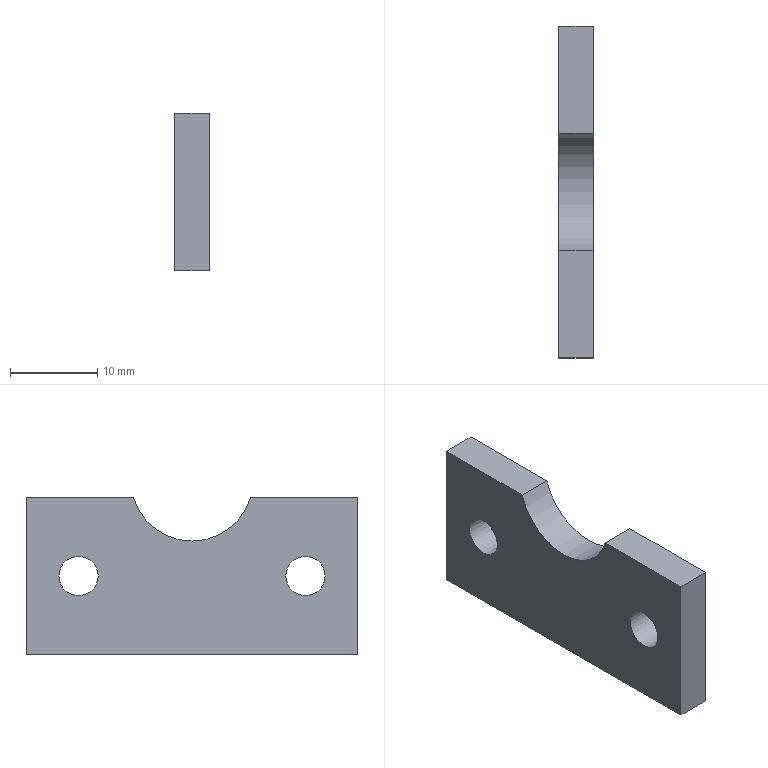Component | NX | BAFFLE_PLATE | 1 solid | 10 faces | box 4 x 38 x 18 mm | volume 2411 mm3 | plane 7 | cylinder 3 | commonest cylinder face diameters 4.5 x2 14 x1
STEP:
#1=CARTESIAN_POINT('',(0.,0.,0.));
#2=DIRECTION('',(0.,0.,1.));
#3=DIRECTION('',(1.,0.,0.));
#4=AXIS2_PLACEMENT_3D('',#1,#2,#3);
#5=CARTESIAN_POINT('',(-20.,-19.,34.5));
#6=VERTEX_POINT('',#5);
#7=CARTESIAN_POINT('',(-20.,-19.,16.5));
#8=VERTEX_POINT('',#7);
#9=CARTESIAN_POINT('',(-20.,-19.,34.5));
#10=DIRECTION('',(0.,0.,-1.));
#11=VECTOR('',#10,1.);
#12=LINE('',#9,#11);
#13=CARTESIAN_POINT('',(-16.,-19.,34.5));
#14=DIRECTION('',(0.,1.,0.));
#15=DIRECTION('',(0.,0.,1.));
#16=AXIS2_PLACEMENT_3D('',#13,#14,#15);
#17=PLANE('',#16);
#18=CARTESIAN_POINT('',(0.,-4.));
#19=DIRECTION('',(-1.,0.));
#20=VECTOR('',#19,1.);
#21=LINE('',#18,#20);
#22=(GEOMETRIC_REPRESENTATION_CONTEXT(2)PARAMETRIC_REPRESENTATION_CONTEXT()REPRESENTATION_CONTEXT('',''));
#23=DEFINITIONAL_REPRESENTATION('',(#21),#22);
#24=PCURVE('',#17,#23);
#25=CARTESIAN_POINT('',(-20.,0.,36.5));
#26=DIRECTION('',(-1.,0.,0.));
#27=DIRECTION('',(0.,0.,1.));
#28=AXIS2_PLACEMENT_3D('',#25,#26,#27);
#29=PLANE('',#28);
#30=CARTESIAN_POINT('',(-2.,-19.));
#31=DIRECTION('',(-1.,0.));
#32=VECTOR('',#31,1.);
#33=LINE('',#30,#32);
#34=(GEOMETRIC_REPRESENTATION_CONTEXT(2)PARAMETRIC_REPRESENTATION_CONTEXT()REPRESENTATION_CONTEXT('',''));
#35=DEFINITIONAL_REPRESENTATION('',(#33),#34);
#36=PCURVE('',#29,#35);
#37=SURFACE_CURVE('',#12,(#24,#36),.PCURVE_S1.);
#38=EDGE_CURVE('',#6,#8,#37,.T.);
#39=ORIENTED_EDGE('',*,*,#38,.T.);
#40=CARTESIAN_POINT('',(-16.,-19.,16.5));
#41=VERTEX_POINT('',#40);
#42=CARTESIAN_POINT('',(-16.,-19.,16.5));
#43=DIRECTION('',(-1.,0.,0.));
#44=VECTOR('',#43,1.);
#45=LINE('',#42,#44);
#46=CARTESIAN_POINT('',(-18.,0.));
#47=DIRECTION('',(0.,-1.));
#48=VECTOR('',#47,1.);
#49=LINE('',#46,#48);
#50=(GEOMETRIC_REPRESENTATION_CONTEXT(2)PARAMETRIC_REPRESENTATION_CONTEXT()REPRESENTATION_CONTEXT('',''));
#51=DEFINITIONAL_REPRESENTATION('',(#49),#50);
#52=PCURVE('',#17,#51);
#53=CARTESIAN_POINT('',(-16.,-19.,16.5));
#54=DIRECTION('',(0.,0.,1.));
#55=DIRECTION('',(1.,0.,0.));
#56=AXIS2_PLACEMENT_3D('',#53,#54,#55);
#57=PLANE('',#56);
#58=CARTESIAN_POINT('',(0.,0.));
#59=DIRECTION('',(-1.,0.));
#60=VECTOR('',#59,1.);
#61=LINE('',#58,#60);
#62=(GEOMETRIC_REPRESENTATION_CONTEXT(2)PARAMETRIC_REPRESENTATION_CONTEXT()REPRESENTATION_CONTEXT('',''));
#63=DEFINITIONAL_REPRESENTATION('',(#61),#62);
#64=PCURVE('',#57,#63);
#65=SURFACE_CURVE('',#45,(#52,#64),.PCURVE_S1.);
#66=EDGE_CURVE('',#41,#8,#65,.T.);
#67=ORIENTED_EDGE('',*,*,#66,.F.);
#68=CARTESIAN_POINT('',(-16.,-19.,34.5));
#69=VERTEX_POINT('',#68);
#70=CARTESIAN_POINT('',(-16.,-19.,34.5));
#71=DIRECTION('',(0.,0.,-1.));
#72=VECTOR('',#71,1.);
#73=LINE('',#70,#72);
#74=CARTESIAN_POINT('',(0.,0.));
#75=DIRECTION('',(-1.,0.));
#76=VECTOR('',#75,1.);
#77=LINE('',#74,#76);
#78=(GEOMETRIC_REPRESENTATION_CONTEXT(2)PARAMETRIC_REPRESENTATION_CONTEXT()REPRESENTATION_CONTEXT('',''));
#79=DEFINITIONAL_REPRESENTATION('',(#77),#78);
#80=PCURVE('',#17,#79);
#81=CARTESIAN_POINT('',(-16.,0.,36.5));
#82=DIRECTION('',(-1.,0.,0.));
#83=DIRECTION('',(0.,0.,1.));
#84=AXIS2_PLACEMENT_3D('',#81,#82,#83);
#85=PLANE('',#84);
#86=CARTESIAN_POINT('',(-2.,-19.));
#87=DIRECTION('',(-1.,0.));
#88=VECTOR('',#87,1.);
#89=LINE('',#86,#88);
#90=(GEOMETRIC_REPRESENTATION_CONTEXT(2)PARAMETRIC_REPRESENTATION_CONTEXT()REPRESENTATION_CONTEXT('',''));
#91=DEFINITIONAL_REPRESENTATION('',(#89),#90);
#92=PCURVE('',#85,#91);
#93=SURFACE_CURVE('',#73,(#80,#92),.PCURVE_S1.);
#94=EDGE_CURVE('',#69,#41,#93,.T.);
#95=ORIENTED_EDGE('',*,*,#94,.F.);
#96=CARTESIAN_POINT('',(-16.,-19.,34.5));
#97=DIRECTION('',(-1.,0.,0.));
#98=VECTOR('',#97,1.);
#99=LINE('',#96,#98);
#100=CARTESIAN_POINT('',(0.,0.));
#101=DIRECTION('',(0.,-1.));
#102=VECTOR('',#101,1.);
#103=LINE('',#100,#102);
#104=(GEOMETRIC_REPRESENTATION_CONTEXT(2)PARAMETRIC_REPRESENTATION_CONTEXT()REPRESENTATION_CONTEXT('',''));
#105=DEFINITIONAL_REPRESENTATION('',(#103),#104);
#106=PCURVE('',#17,#105);
#107=CARTESIAN_POINT('',(-16.,-6.708,34.5));
#108=DIRECTION('',(0.,0.,-1.));
#109=DIRECTION('',(-1.,0.,0.));
#110=AXIS2_PLACEMENT_3D('',#107,#108,#109);
#111=PLANE('',#110);
#112=CARTESIAN_POINT('',(0.,-12.292));
#113=DIRECTION('',(1.,0.));
#114=VECTOR('',#113,1.);
#115=LINE('',#112,#114);
#116=(GEOMETRIC_REPRESENTATION_CONTEXT(2)PARAMETRIC_REPRESENTATION_CONTEXT()REPRESENTATION_CONTEXT('',''));
#117=DEFINITIONAL_REPRESENTATION('',(#115),#116);
#118=PCURVE('',#111,#117);
#119=SURFACE_CURVE('',#99,(#106,#118),.PCURVE_S1.);
#120=EDGE_CURVE('',#69,#6,#119,.T.);
#121=ORIENTED_EDGE('',*,*,#120,.T.);
#122=EDGE_LOOP('',(#39,#67,#95,#121));
#123=FACE_BOUND('',#122,.T.);
#124=ADVANCED_FACE('',(#123),#17,.F.);
#125=CARTESIAN_POINT('',(-20.,19.,16.5));
#126=VERTEX_POINT('',#125);
#127=CARTESIAN_POINT('',(-20.,-19.,16.5));
#128=DIRECTION('',(0.,1.,0.));
#129=VECTOR('',#128,1.);
#130=LINE('',#127,#129);
#131=CARTESIAN_POINT('',(-4.,0.));
#132=DIRECTION('',(0.,1.));
#133=VECTOR('',#132,1.);
#134=LINE('',#131,#133);
#135=(GEOMETRIC_REPRESENTATION_CONTEXT(2)PARAMETRIC_REPRESENTATION_CONTEXT()REPRESENTATION_CONTEXT('',''));
#136=DEFINITIONAL_REPRESENTATION('',(#134),#135);
#137=PCURVE('',#57,#136);
#138=CARTESIAN_POINT('',(-20.,-19.));
#139=DIRECTION('',(0.,1.));
#140=VECTOR('',#139,1.);
#141=LINE('',#138,#140);
#142=(GEOMETRIC_REPRESENTATION_CONTEXT(2)PARAMETRIC_REPRESENTATION_CONTEXT()REPRESENTATION_CONTEXT('',''));
#143=DEFINITIONAL_REPRESENTATION('',(#141),#142);
#144=PCURVE('',#29,#143);
#145=SURFACE_CURVE('',#130,(#137,#144),.PCURVE_S1.);
#146=EDGE_CURVE('',#8,#126,#145,.T.);
#147=ORIENTED_EDGE('',*,*,#146,.T.);
#148=CARTESIAN_POINT('',(-16.,19.,16.5));
#149=VERTEX_POINT('',#148);
#150=CARTESIAN_POINT('',(-16.,19.,16.5));
#151=DIRECTION('',(-1.,0.,0.));
#152=VECTOR('',#151,1.);
#153=LINE('',#150,#152);
#154=CARTESIAN_POINT('',(0.,38.));
#155=DIRECTION('',(-1.,0.));
#156=VECTOR('',#155,1.);
#157=LINE('',#154,#156);
#158=(GEOMETRIC_REPRESENTATION_CONTEXT(2)PARAMETRIC_REPRESENTATION_CONTEXT()REPRESENTATION_CONTEXT('',''));
#159=DEFINITIONAL_REPRESENTATION('',(#157),#158);
#160=PCURVE('',#57,#159);
#161=CARTESIAN_POINT('',(-16.,19.,16.5));
#162=DIRECTION('',(0.,-1.,0.));
#163=DIRECTION('',(0.,0.,-1.));
#164=AXIS2_PLACEMENT_3D('',#161,#162,#163);
#165=PLANE('',#164);
#166=CARTESIAN_POINT('',(0.,0.));
#167=DIRECTION('',(0.,-1.));
#168=VECTOR('',#167,1.);
#169=LINE('',#166,#168);
#170=(GEOMETRIC_REPRESENTATION_CONTEXT(2)PARAMETRIC_REPRESENTATION_CONTEXT()REPRESENTATION_CONTEXT('',''));
#171=DEFINITIONAL_REPRESENTATION('',(#169),#170);
#172=PCURVE('',#165,#171);
#173=SURFACE_CURVE('',#153,(#160,#172),.PCURVE_S1.);
#174=EDGE_CURVE('',#149,#126,#173,.T.);
#175=ORIENTED_EDGE('',*,*,#174,.F.);
#176=CARTESIAN_POINT('',(-16.,-19.,16.5));
#177=DIRECTION('',(0.,1.,0.));
#178=VECTOR('',#177,1.);
#179=LINE('',#176,#178);
#180=CARTESIAN_POINT('',(0.,0.));
#181=DIRECTION('',(0.,1.));
#182=VECTOR('',#181,1.);
#183=LINE('',#180,#182);
#184=(GEOMETRIC_REPRESENTATION_CONTEXT(2)PARAMETRIC_REPRESENTATION_CONTEXT()REPRESENTATION_CONTEXT('',''));
#185=DEFINITIONAL_REPRESENTATION('',(#183),#184);
#186=PCURVE('',#57,#185);
#187=CARTESIAN_POINT('',(-20.,-19.));
#188=DIRECTION('',(0.,1.));
#189=VECTOR('',#188,1.);
#190=LINE('',#187,#189);
#191=(GEOMETRIC_REPRESENTATION_CONTEXT(2)PARAMETRIC_REPRESENTATION_CONTEXT()REPRESENTATION_CONTEXT('',''));
#192=DEFINITIONAL_REPRESENTATION('',(#190),#191);
#193=PCURVE('',#85,#192);
#194=SURFACE_CURVE('',#179,(#186,#193),.PCURVE_S1.);
#195=EDGE_CURVE('',#41,#149,#194,.T.);
#196=ORIENTED_EDGE('',*,*,#195,.F.);
#197=ORIENTED_EDGE('',*,*,#66,.T.);
#198=EDGE_LOOP('',(#147,#175,#196,#197));
#199=FACE_BOUND('',#198,.T.);
#200=ADVANCED_FACE('',(#199),#57,.F.);
#201=CARTESIAN_POINT('',(-20.,19.,34.5));
#202=VERTEX_POINT('',#201);
#203=CARTESIAN_POINT('',(-20.,19.,16.5));
#204=DIRECTION('',(0.,0.,1.));
#205=VECTOR('',#204,1.);
#206=LINE('',#203,#205);
#207=CARTESIAN_POINT('',(0.,-4.));
#208=DIRECTION('',(-1.,0.));
#209=VECTOR('',#208,1.);
#210=LINE('',#207,#209);
#211=(GEOMETRIC_REPRESENTATION_CONTEXT(2)PARAMETRIC_REPRESENTATION_CONTEXT()REPRESENTATION_CONTEXT('',''));
#212=DEFINITIONAL_REPRESENTATION('',(#210),#211);
#213=PCURVE('',#165,#212);
#214=CARTESIAN_POINT('',(-20.,19.));
#215=DIRECTION('',(1.,0.));
#216=VECTOR('',#215,1.);
#217=LINE('',#214,#216);
#218=(GEOMETRIC_REPRESENTATION_CONTEXT(2)PARAMETRIC_REPRESENTATION_CONTEXT()REPRESENTATION_CONTEXT('',''));
#219=DEFINITIONAL_REPRESENTATION('',(#217),#218);
#220=PCURVE('',#29,#219);
#221=SURFACE_CURVE('',#206,(#213,#220),.PCURVE_S1.);
#222=EDGE_CURVE('',#126,#202,#221,.T.);
#223=ORIENTED_EDGE('',*,*,#222,.T.);
#224=CARTESIAN_POINT('',(-16.,19.,34.5));
#225=VERTEX_POINT('',#224);
#226=CARTESIAN_POINT('',(-16.,19.,34.5));
#227=DIRECTION('',(-1.,0.,0.));
#228=VECTOR('',#227,1.);
#229=LINE('',#226,#228);
#230=CARTESIAN_POINT('',(-18.,0.));
#231=DIRECTION('',(0.,-1.));
#232=VECTOR('',#231,1.);
#233=LINE('',#230,#232);
#234=(GEOMETRIC_REPRESENTATION_CONTEXT(2)PARAMETRIC_REPRESENTATION_CONTEXT()REPRESENTATION_CONTEXT('',''));
#235=DEFINITIONAL_REPRESENTATION('',(#233),#234);
#236=PCURVE('',#165,#235);
#237=CARTESIAN_POINT('',(-16.,19.,34.5));
#238=DIRECTION('',(0.,0.,-1.));
#239=DIRECTION('',(-1.,0.,0.));
#240=AXIS2_PLACEMENT_3D('',#237,#238,#239);
#241=PLANE('',#240);
#242=CARTESIAN_POINT('',(0.,0.));
#243=DIRECTION('',(1.,0.));
#244=VECTOR('',#243,1.);
#245=LINE('',#242,#244);
#246=(GEOMETRIC_REPRESENTATION_CONTEXT(2)PARAMETRIC_REPRESENTATION_CONTEXT()REPRESENTATION_CONTEXT('',''));
#247=DEFINITIONAL_REPRESENTATION('',(#245),#246);
#248=PCURVE('',#241,#247);
#249=SURFACE_CURVE('',#229,(#236,#248),.PCURVE_S1.);
#250=EDGE_CURVE('',#225,#202,#249,.T.);
#251=ORIENTED_EDGE('',*,*,#250,.F.);
#252=CARTESIAN_POINT('',(-16.,19.,16.5));
#253=DIRECTION('',(0.,0.,1.));
#254=VECTOR('',#253,1.);
#255=LINE('',#252,#254);
#256=CARTESIAN_POINT('',(0.,0.));
#257=DIRECTION('',(-1.,0.));
#258=VECTOR('',#257,1.);
#259=LINE('',#256,#258);
#260=(GEOMETRIC_REPRESENTATION_CONTEXT(2)PARAMETRIC_REPRESENTATION_CONTEXT()REPRESENTATION_CONTEXT('',''));
#261=DEFINITIONAL_REPRESENTATION('',(#259),#260);
#262=PCURVE('',#165,#261);
#263=CARTESIAN_POINT('',(-20.,19.));
#264=DIRECTION('',(1.,0.));
#265=VECTOR('',#264,1.);
#266=LINE('',#263,#265);
#267=(GEOMETRIC_REPRESENTATION_CONTEXT(2)PARAMETRIC_REPRESENTATION_CONTEXT()REPRESENTATION_CONTEXT('',''));
#268=DEFINITIONAL_REPRESENTATION('',(#266),#267);
#269=PCURVE('',#85,#268);
#270=SURFACE_CURVE('',#255,(#262,#269),.PCURVE_S1.);
#271=EDGE_CURVE('',#149,#225,#270,.T.);
#272=ORIENTED_EDGE('',*,*,#271,.F.);
#273=ORIENTED_EDGE('',*,*,#174,.T.);
#274=EDGE_LOOP('',(#223,#251,#272,#273));
#275=FACE_BOUND('',#274,.T.);
#276=ADVANCED_FACE('',(#275),#165,.F.);
#277=CARTESIAN_POINT('',(-20.,6.708,34.5));
#278=VERTEX_POINT('',#277);
#279=CARTESIAN_POINT('',(-20.,19.,34.5));
#280=DIRECTION('',(0.,-1.,0.));
#281=VECTOR('',#280,1.);
#282=LINE('',#279,#281);
#283=CARTESIAN_POINT('',(4.,0.));
#284=DIRECTION('',(0.,-1.));
#285=VECTOR('',#284,1.);
#286=LINE('',#283,#285);
#287=(GEOMETRIC_REPRESENTATION_CONTEXT(2)PARAMETRIC_REPRESENTATION_CONTEXT()REPRESENTATION_CONTEXT('',''));
#288=DEFINITIONAL_REPRESENTATION('',(#286),#287);
#289=PCURVE('',#241,#288);
#290=CARTESIAN_POINT('',(-2.,19.));
#291=DIRECTION('',(0.,-1.));
#292=VECTOR('',#291,1.);
#293=LINE('',#290,#292);
#294=(GEOMETRIC_REPRESENTATION_CONTEXT(2)PARAMETRIC_REPRESENTATION_CONTEXT()REPRESENTATION_CONTEXT('',''));
#295=DEFINITIONAL_REPRESENTATION('',(#293),#294);
#296=PCURVE('',#29,#295);
#297=SURFACE_CURVE('',#282,(#289,#296),.PCURVE_S1.);
#298=EDGE_CURVE('',#202,#278,#297,.T.);
#299=ORIENTED_EDGE('',*,*,#298,.T.);
#300=CARTESIAN_POINT('',(-16.,6.708,34.5));
#301=VERTEX_POINT('',#300);
#302=CARTESIAN_POINT('',(-16.,6.708,34.5));
#303=DIRECTION('',(-1.,0.,0.));
#304=VECTOR('',#303,1.);
#305=LINE('',#302,#304);
#306=CARTESIAN_POINT('',(0.,-12.292));
#307=DIRECTION('',(1.,0.));
#308=VECTOR('',#307,1.);
#309=LINE('',#306,#308);
#310=(GEOMETRIC_REPRESENTATION_CONTEXT(2)PARAMETRIC_REPRESENTATION_CONTEXT()REPRESENTATION_CONTEXT('',''));
#311=DEFINITIONAL_REPRESENTATION('',(#309),#310);
#312=PCURVE('',#241,#311);
#313=CARTESIAN_POINT('',(-16.,0.,36.5));
#314=DIRECTION('',(-1.,0.,0.));
#315=DIRECTION('',(0.,0.,1.));
#316=AXIS2_PLACEMENT_3D('',#313,#314,#315);
#317=CYLINDRICAL_SURFACE('',#316,7.);
#318=CARTESIAN_POINT('',(1.861,0.));
#319=DIRECTION('',(0.,1.));
#320=VECTOR('',#319,1.);
#321=LINE('',#318,#320);
#322=(GEOMETRIC_REPRESENTATION_CONTEXT(2)PARAMETRIC_REPRESENTATION_CONTEXT()REPRESENTATION_CONTEXT('',''));
#323=DEFINITIONAL_REPRESENTATION('',(#321),#322);
#324=PCURVE('',#317,#323);
#325=SURFACE_CURVE('',#305,(#312,#324),.PCURVE_S1.);
#326=EDGE_CURVE('',#301,#278,#325,.T.);
#327=ORIENTED_EDGE('',*,*,#326,.F.);
#328=CARTESIAN_POINT('',(-16.,19.,34.5));
#329=DIRECTION('',(0.,-1.,0.));
#330=VECTOR('',#329,1.);
#331=LINE('',#328,#330);
#332=CARTESIAN_POINT('',(0.,0.));
#333=DIRECTION('',(0.,-1.));
#334=VECTOR('',#333,1.);
#335=LINE('',#332,#334);
#336=(GEOMETRIC_REPRESENTATION_CONTEXT(2)PARAMETRIC_REPRESENTATION_CONTEXT()REPRESENTATION_CONTEXT('',''));
#337=DEFINITIONAL_REPRESENTATION('',(#335),#336);
#338=PCURVE('',#241,#337);
#339=CARTESIAN_POINT('',(-2.,19.));
#340=DIRECTION('',(0.,-1.));
#341=VECTOR('',#340,1.);
#342=LINE('',#339,#341);
#343=(GEOMETRIC_REPRESENTATION_CONTEXT(2)PARAMETRIC_REPRESENTATION_CONTEXT()REPRESENTATION_CONTEXT('',''));
#344=DEFINITIONAL_REPRESENTATION('',(#342),#343);
#345=PCURVE('',#85,#344);
#346=SURFACE_CURVE('',#331,(#338,#345),.PCURVE_S1.);
#347=EDGE_CURVE('',#225,#301,#346,.T.);
#348=ORIENTED_EDGE('',*,*,#347,.F.);
#349=ORIENTED_EDGE('',*,*,#250,.T.);
#350=EDGE_LOOP('',(#299,#327,#348,#349));
#351=FACE_BOUND('',#350,.T.);
#352=ADVANCED_FACE('',(#351),#241,.F.);
#353=ORIENTED_EDGE('',*,*,#326,.F.);
#354=CARTESIAN_POINT('',(-16.,-6.708,34.5));
#355=VERTEX_POINT('',#354);
#356=CARTESIAN_POINT('',(-16.,0.,36.5));
#357=DIRECTION('',(-1.,0.,0.));
#358=DIRECTION('',(0.,1.,0.));
#359=AXIS2_PLACEMENT_3D('',#356,#357,#358);
#360=CIRCLE('',#359,7.);
#361=CARTESIAN_POINT('',(1.571,0.));
#362=DIRECTION('',(1.,0.));
#363=VECTOR('',#362,1.);
#364=LINE('',#361,#363);
#365=(GEOMETRIC_REPRESENTATION_CONTEXT(2)PARAMETRIC_REPRESENTATION_CONTEXT()REPRESENTATION_CONTEXT('',''));
#366=DEFINITIONAL_REPRESENTATION('',(#364),#365);
#367=PCURVE('',#317,#366);
#368=CARTESIAN_POINT('',(0.,0.));
#369=DIRECTION('',(0.,1.));
#370=AXIS2_PLACEMENT_2D('',#368,#369);
#371=CIRCLE('',#370,7.);
#372=(GEOMETRIC_REPRESENTATION_CONTEXT(2)PARAMETRIC_REPRESENTATION_CONTEXT()REPRESENTATION_CONTEXT('',''));
#373=DEFINITIONAL_REPRESENTATION('',(#371),#372);
#374=PCURVE('',#85,#373);
#375=SURFACE_CURVE('',#360,(#367,#374),.PCURVE_S1.);
#376=EDGE_CURVE('',#301,#355,#375,.T.);
#377=ORIENTED_EDGE('',*,*,#376,.T.);
#378=CARTESIAN_POINT('',(-20.,-6.708,34.5));
#379=VERTEX_POINT('',#378);
#380=CARTESIAN_POINT('',(-16.,-6.708,34.5));
#381=DIRECTION('',(-1.,0.,0.));
#382=VECTOR('',#381,1.);
#383=LINE('',#380,#382);
#384=CARTESIAN_POINT('',(4.423,0.));
#385=DIRECTION('',(0.,1.));
#386=VECTOR('',#385,1.);
#387=LINE('',#384,#386);
#388=(GEOMETRIC_REPRESENTATION_CONTEXT(2)PARAMETRIC_REPRESENTATION_CONTEXT()REPRESENTATION_CONTEXT('',''));
#389=DEFINITIONAL_REPRESENTATION('',(#387),#388);
#390=PCURVE('',#317,#389);
#391=CARTESIAN_POINT('',(0.,-0.));
#392=DIRECTION('',(1.,0.));
#393=VECTOR('',#392,1.);
#394=LINE('',#391,#393);
#395=(GEOMETRIC_REPRESENTATION_CONTEXT(2)PARAMETRIC_REPRESENTATION_CONTEXT()REPRESENTATION_CONTEXT('',''));
#396=DEFINITIONAL_REPRESENTATION('',(#394),#395);
#397=PCURVE('',#111,#396);
#398=SURFACE_CURVE('',#383,(#390,#397),.PCURVE_S1.);
#399=EDGE_CURVE('',#355,#379,#398,.T.);
#400=ORIENTED_EDGE('',*,*,#399,.T.);
#401=CARTESIAN_POINT('',(-20.,0.,36.5));
#402=DIRECTION('',(-1.,0.,0.));
#403=DIRECTION('',(0.,1.,0.));
#404=AXIS2_PLACEMENT_3D('',#401,#402,#403);
#405=CIRCLE('',#404,7.);
#406=CARTESIAN_POINT('',(1.571,4.));
#407=DIRECTION('',(1.,0.));
#408=VECTOR('',#407,1.);
#409=LINE('',#406,#408);
#410=(GEOMETRIC_REPRESENTATION_CONTEXT(2)PARAMETRIC_REPRESENTATION_CONTEXT()REPRESENTATION_CONTEXT('',''));
#411=DEFINITIONAL_REPRESENTATION('',(#409),#410);
#412=PCURVE('',#317,#411);
#413=CARTESIAN_POINT('',(0.,0.));
#414=DIRECTION('',(0.,1.));
#415=AXIS2_PLACEMENT_2D('',#413,#414);
#416=CIRCLE('',#415,7.);
#417=(GEOMETRIC_REPRESENTATION_CONTEXT(2)PARAMETRIC_REPRESENTATION_CONTEXT()REPRESENTATION_CONTEXT('',''));
#418=DEFINITIONAL_REPRESENTATION('',(#416),#417);
#419=PCURVE('',#29,#418);
#420=SURFACE_CURVE('',#405,(#412,#419),.PCURVE_S1.);
#421=EDGE_CURVE('',#278,#379,#420,.T.);
#422=ORIENTED_EDGE('',*,*,#421,.F.);
#423=EDGE_LOOP('',(#353,#377,#400,#422));
#424=FACE_BOUND('',#423,.F.);
#425=ADVANCED_FACE('',(#424),#317,.F.);
#426=CARTESIAN_POINT('',(-16.,10.75,25.5));
#427=VERTEX_POINT('',#426);
#428=CARTESIAN_POINT('',(-16.,13.,25.5));
#429=DIRECTION('',(-1.,0.,0.));
#430=DIRECTION('',(0.,-1.,0.));
#431=AXIS2_PLACEMENT_3D('',#428,#429,#430);
#432=CIRCLE('',#431,2.25);
#433=CARTESIAN_POINT('',(-16.,13.,25.5));
#434=DIRECTION('',(-1.,0.,0.));
#435=DIRECTION('',(0.,0.,1.));
#436=AXIS2_PLACEMENT_3D('',#433,#434,#435);
#437=CYLINDRICAL_SURFACE('',#436,2.25);
#438=CARTESIAN_POINT('',(4.712,0.));
#439=DIRECTION('',(1.,0.));
#440=VECTOR('',#439,1.);
#441=LINE('',#438,#440);
#442=(GEOMETRIC_REPRESENTATION_CONTEXT(2)PARAMETRIC_REPRESENTATION_CONTEXT()REPRESENTATION_CONTEXT('',''));
#443=DEFINITIONAL_REPRESENTATION('',(#441),#442);
#444=PCURVE('',#437,#443);
#445=CARTESIAN_POINT('',(-11.,13.));
#446=DIRECTION('',(0.,-1.));
#447=AXIS2_PLACEMENT_2D('',#445,#446);
#448=CIRCLE('',#447,2.25);
#449=(GEOMETRIC_REPRESENTATION_CONTEXT(2)PARAMETRIC_REPRESENTATION_CONTEXT()REPRESENTATION_CONTEXT('',''));
#450=DEFINITIONAL_REPRESENTATION('',(#448),#449);
#451=PCURVE('',#85,#450);
#452=SURFACE_CURVE('',#432,(#444,#451),.PCURVE_S1.);
#453=EDGE_CURVE('',#427,#427,#452,.T.);
#454=ORIENTED_EDGE('',*,*,#453,.T.);
#455=CARTESIAN_POINT('',(-20.,10.75,25.5));
#456=VERTEX_POINT('',#455);
#457=CARTESIAN_POINT('',(-16.,10.75,25.5));
#458=CARTESIAN_POINT('',(-20.,10.75,25.5));
#459=B_SPLINE_CURVE_WITH_KNOTS('',1,(#457,#458),.UNSPECIFIED.,.F.,.F.,(2,2),(0.,4.),.PIECEWISE_BEZIER_KNOTS.);
#460=CARTESIAN_POINT('',(10.996,0.));
#461=DIRECTION('',(0.,1.));
#462=VECTOR('',#461,1.);
#463=LINE('',#460,#462);
#464=(GEOMETRIC_REPRESENTATION_CONTEXT(2)PARAMETRIC_REPRESENTATION_CONTEXT()REPRESENTATION_CONTEXT('',''));
#465=DEFINITIONAL_REPRESENTATION('',(#463),#464);
#466=PCURVE('',#437,#465);
#467=CARTESIAN_POINT('',(4.712,0.));
#468=DIRECTION('',(0.,1.));
#469=VECTOR('',#468,1.);
#470=LINE('',#467,#469);
#471=(GEOMETRIC_REPRESENTATION_CONTEXT(2)PARAMETRIC_REPRESENTATION_CONTEXT()REPRESENTATION_CONTEXT('',''));
#472=DEFINITIONAL_REPRESENTATION('',(#470),#471);
#473=PCURVE('',#437,#472);
#474=SEAM_CURVE('',#459,(#466,#473),.PCURVE_S1.);
#475=EDGE_CURVE('',#427,#456,#474,.T.);
#476=ORIENTED_EDGE('',*,*,#475,.T.);
#477=CARTESIAN_POINT('',(-20.,13.,25.5));
#478=DIRECTION('',(-1.,0.,0.));
#479=DIRECTION('',(0.,-1.,0.));
#480=AXIS2_PLACEMENT_3D('',#477,#478,#479);
#481=CIRCLE('',#480,2.25);
#482=CARTESIAN_POINT('',(4.712,4.));
#483=DIRECTION('',(1.,0.));
#484=VECTOR('',#483,1.);
#485=LINE('',#482,#484);
#486=(GEOMETRIC_REPRESENTATION_CONTEXT(2)PARAMETRIC_REPRESENTATION_CONTEXT()REPRESENTATION_CONTEXT('',''));
#487=DEFINITIONAL_REPRESENTATION('',(#485),#486);
#488=PCURVE('',#437,#487);
#489=CARTESIAN_POINT('',(-11.,13.));
#490=DIRECTION('',(0.,-1.));
#491=AXIS2_PLACEMENT_2D('',#489,#490);
#492=CIRCLE('',#491,2.25);
#493=(GEOMETRIC_REPRESENTATION_CONTEXT(2)PARAMETRIC_REPRESENTATION_CONTEXT()REPRESENTATION_CONTEXT('',''));
#494=DEFINITIONAL_REPRESENTATION('',(#492),#493);
#495=PCURVE('',#29,#494);
#496=SURFACE_CURVE('',#481,(#488,#495),.PCURVE_S1.);
#497=EDGE_CURVE('',#456,#456,#496,.T.);
#498=ORIENTED_EDGE('',*,*,#497,.F.);
#499=ORIENTED_EDGE('',*,*,#475,.F.);
#500=EDGE_LOOP('',(#454,#476,#498,#499));
#501=FACE_BOUND('',#500,.F.);
#502=ADVANCED_FACE('',(#501),#437,.F.);
#503=CARTESIAN_POINT('',(-20.,-6.708,34.5));
#504=DIRECTION('',(0.,-1.,0.));
#505=VECTOR('',#504,1.);
#506=LINE('',#503,#505);
#507=CARTESIAN_POINT('',(4.,0.));
#508=DIRECTION('',(0.,-1.));
#509=VECTOR('',#508,1.);
#510=LINE('',#507,#509);
#511=(GEOMETRIC_REPRESENTATION_CONTEXT(2)PARAMETRIC_REPRESENTATION_CONTEXT()REPRESENTATION_CONTEXT('',''));
#512=DEFINITIONAL_REPRESENTATION('',(#510),#511);
#513=PCURVE('',#111,#512);
#514=CARTESIAN_POINT('',(-2.,-6.708));
#515=DIRECTION('',(0.,-1.));
#516=VECTOR('',#515,1.);
#517=LINE('',#514,#516);
#518=(GEOMETRIC_REPRESENTATION_CONTEXT(2)PARAMETRIC_REPRESENTATION_CONTEXT()REPRESENTATION_CONTEXT('',''));
#519=DEFINITIONAL_REPRESENTATION('',(#517),#518);
#520=PCURVE('',#29,#519);
#521=SURFACE_CURVE('',#506,(#513,#520),.PCURVE_S1.);
#522=EDGE_CURVE('',#379,#6,#521,.T.);
#523=ORIENTED_EDGE('',*,*,#522,.T.);
#524=ORIENTED_EDGE('',*,*,#120,.F.);
#525=CARTESIAN_POINT('',(-16.,-6.708,34.5));
#526=DIRECTION('',(0.,-1.,0.));
#527=VECTOR('',#526,1.);
#528=LINE('',#525,#527);
#529=CARTESIAN_POINT('',(0.,0.));
#530=DIRECTION('',(0.,-1.));
#531=VECTOR('',#530,1.);
#532=LINE('',#529,#531);
#533=(GEOMETRIC_REPRESENTATION_CONTEXT(2)PARAMETRIC_REPRESENTATION_CONTEXT()REPRESENTATION_CONTEXT('',''));
#534=DEFINITIONAL_REPRESENTATION('',(#532),#533);
#535=PCURVE('',#111,#534);
#536=CARTESIAN_POINT('',(-2.,-6.708));
#537=DIRECTION('',(0.,-1.));
#538=VECTOR('',#537,1.);
#539=LINE('',#536,#538);
#540=(GEOMETRIC_REPRESENTATION_CONTEXT(2)PARAMETRIC_REPRESENTATION_CONTEXT()REPRESENTATION_CONTEXT('',''));
#541=DEFINITIONAL_REPRESENTATION('',(#539),#540);
#542=PCURVE('',#85,#541);
#543=SURFACE_CURVE('',#528,(#535,#542),.PCURVE_S1.);
#544=EDGE_CURVE('',#355,#69,#543,.T.);
#545=ORIENTED_EDGE('',*,*,#544,.F.);
#546=ORIENTED_EDGE('',*,*,#399,.T.);
#547=EDGE_LOOP('',(#523,#524,#545,#546));
#548=FACE_BOUND('',#547,.T.);
#549=ADVANCED_FACE('',(#548),#111,.F.);
#550=CARTESIAN_POINT('',(-16.,-10.75,25.5));
#551=VERTEX_POINT('',#550);
#552=CARTESIAN_POINT('',(-16.,-13.,25.5));
#553=DIRECTION('',(1.,0.,0.));
#554=DIRECTION('',(0.,1.,0.));
#555=AXIS2_PLACEMENT_3D('',#552,#553,#554);
#556=CIRCLE('',#555,2.25);
#557=CARTESIAN_POINT('',(-16.,-13.,25.5));
#558=DIRECTION('',(-1.,0.,0.));
#559=DIRECTION('',(0.,0.,1.));
#560=AXIS2_PLACEMENT_3D('',#557,#558,#559);
#561=CYLINDRICAL_SURFACE('',#560,2.25);
#562=CARTESIAN_POINT('',(7.854,0.));
#563=DIRECTION('',(-1.,0.));
#564=VECTOR('',#563,1.);
#565=LINE('',#562,#564);
#566=(GEOMETRIC_REPRESENTATION_CONTEXT(2)PARAMETRIC_REPRESENTATION_CONTEXT()REPRESENTATION_CONTEXT('',''));
#567=DEFINITIONAL_REPRESENTATION('',(#565),#566);
#568=PCURVE('',#561,#567);
#569=CARTESIAN_POINT('',(-11.,-10.75));
#570=CARTESIAN_POINT('',(-7.103,-10.75));
#571=CARTESIAN_POINT('',(-9.051,-14.125));
#572=CARTESIAN_POINT('',(-11.,-17.5));
#573=CARTESIAN_POINT('',(-12.949,-14.125));
#574=CARTESIAN_POINT('',(-14.897,-10.75));
#575=CARTESIAN_POINT('',(-11.,-10.75));
#576=(BOUNDED_CURVE()B_SPLINE_CURVE(2,(#569,#570,#571,#572,#573,#574,#575),.UNSPECIFIED.,.T.,.F.)B_SPLINE_CURVE_WITH_KNOTS((1,2,2,2,2,1),(-2.094,0.,2.094,4.189,6.283,8.378),.UNSPECIFIED.)CURVE()GEOMETRIC_REPRESENTATION_ITEM()RATIONAL_B_SPLINE_CURVE((1.,0.5,1.,0.5,1.,0.5,1.))REPRESENTATION_ITEM(''));
#577=(GEOMETRIC_REPRESENTATION_CONTEXT(2)PARAMETRIC_REPRESENTATION_CONTEXT()REPRESENTATION_CONTEXT('',''));
#578=DEFINITIONAL_REPRESENTATION('',(#576),#577);
#579=PCURVE('',#85,#578);
#580=SURFACE_CURVE('',#556,(#568,#579),.PCURVE_S1.);
#581=EDGE_CURVE('',#551,#551,#580,.T.);
#582=ORIENTED_EDGE('',*,*,#581,.F.);
#583=CARTESIAN_POINT('',(-20.,-10.75,25.5));
#584=VERTEX_POINT('',#583);
#585=CARTESIAN_POINT('',(-16.,-10.75,25.5));
#586=CARTESIAN_POINT('',(-20.,-10.75,25.5));
#587=B_SPLINE_CURVE_WITH_KNOTS('',1,(#585,#586),.UNSPECIFIED.,.F.,.F.,(2,2),(0.,4.),.PIECEWISE_BEZIER_KNOTS.);
#588=CARTESIAN_POINT('',(7.854,0.));
#589=DIRECTION('',(0.,1.));
#590=VECTOR('',#589,1.);
#591=LINE('',#588,#590);
#592=(GEOMETRIC_REPRESENTATION_CONTEXT(2)PARAMETRIC_REPRESENTATION_CONTEXT()REPRESENTATION_CONTEXT('',''));
#593=DEFINITIONAL_REPRESENTATION('',(#591),#592);
#594=PCURVE('',#561,#593);
#595=CARTESIAN_POINT('',(1.571,0.));
#596=DIRECTION('',(0.,1.));
#597=VECTOR('',#596,1.);
#598=LINE('',#595,#597);
#599=(GEOMETRIC_REPRESENTATION_CONTEXT(2)PARAMETRIC_REPRESENTATION_CONTEXT()REPRESENTATION_CONTEXT('',''));
#600=DEFINITIONAL_REPRESENTATION('',(#598),#599);
#601=PCURVE('',#561,#600);
#602=SEAM_CURVE('',#587,(#594,#601),.PCURVE_S1.);
#603=EDGE_CURVE('',#551,#584,#602,.T.);
#604=ORIENTED_EDGE('',*,*,#603,.T.);
#605=CARTESIAN_POINT('',(-20.,-13.,25.5));
#606=DIRECTION('',(1.,0.,0.));
#607=DIRECTION('',(0.,1.,0.));
#608=AXIS2_PLACEMENT_3D('',#605,#606,#607);
#609=CIRCLE('',#608,2.25);
#610=CARTESIAN_POINT('',(7.854,4.));
#611=DIRECTION('',(-1.,0.));
#612=VECTOR('',#611,1.);
#613=LINE('',#610,#612);
#614=(GEOMETRIC_REPRESENTATION_CONTEXT(2)PARAMETRIC_REPRESENTATION_CONTEXT()REPRESENTATION_CONTEXT('',''));
#615=DEFINITIONAL_REPRESENTATION('',(#613),#614);
#616=PCURVE('',#561,#615);
#617=CARTESIAN_POINT('',(-11.,-10.75));
#618=CARTESIAN_POINT('',(-7.103,-10.75));
#619=CARTESIAN_POINT('',(-9.051,-14.125));
#620=CARTESIAN_POINT('',(-11.,-17.5));
#621=CARTESIAN_POINT('',(-12.949,-14.125));
#622=CARTESIAN_POINT('',(-14.897,-10.75));
#623=CARTESIAN_POINT('',(-11.,-10.75));
#624=(BOUNDED_CURVE()B_SPLINE_CURVE(2,(#617,#618,#619,#620,#621,#622,#623),.UNSPECIFIED.,.T.,.F.)B_SPLINE_CURVE_WITH_KNOTS((1,2,2,2,2,1),(-2.094,0.,2.094,4.189,6.283,8.378),.UNSPECIFIED.)CURVE()GEOMETRIC_REPRESENTATION_ITEM()RATIONAL_B_SPLINE_CURVE((1.,0.5,1.,0.5,1.,0.5,1.))REPRESENTATION_ITEM(''));
#625=(GEOMETRIC_REPRESENTATION_CONTEXT(2)PARAMETRIC_REPRESENTATION_CONTEXT()REPRESENTATION_CONTEXT('',''));
#626=DEFINITIONAL_REPRESENTATION('',(#624),#625);
#627=PCURVE('',#29,#626);
#628=SURFACE_CURVE('',#609,(#616,#627),.PCURVE_S1.);
#629=EDGE_CURVE('',#584,#584,#628,.T.);
#630=ORIENTED_EDGE('',*,*,#629,.T.);
#631=ORIENTED_EDGE('',*,*,#603,.F.);
#632=EDGE_LOOP('',(#582,#604,#630,#631));
#633=FACE_BOUND('',#632,.F.);
#634=ADVANCED_FACE('',(#633),#561,.F.);
#635=ORIENTED_EDGE('',*,*,#94,.T.);
#636=ORIENTED_EDGE('',*,*,#195,.T.);
#637=ORIENTED_EDGE('',*,*,#271,.T.);
#638=ORIENTED_EDGE('',*,*,#347,.T.);
#639=ORIENTED_EDGE('',*,*,#376,.T.);
#640=ORIENTED_EDGE('',*,*,#544,.T.);
#641=EDGE_LOOP('',(#635,#636,#637,#638,#639,#640));
#642=FACE_BOUND('',#641,.T.);
#643=ORIENTED_EDGE('',*,*,#453,.T.);
#644=EDGE_LOOP('',(#643));
#645=FACE_BOUND('',#644,.T.);
#646=ORIENTED_EDGE('',*,*,#581,.F.);
#647=EDGE_LOOP('',(#646));
#648=FACE_BOUND('',#647,.T.);
#649=ADVANCED_FACE('',(#642,#645,#648),#85,.F.);
#650=ORIENTED_EDGE('',*,*,#38,.F.);
#651=ORIENTED_EDGE('',*,*,#522,.F.);
#652=ORIENTED_EDGE('',*,*,#421,.F.);
#653=ORIENTED_EDGE('',*,*,#298,.F.);
#654=ORIENTED_EDGE('',*,*,#222,.F.);
#655=ORIENTED_EDGE('',*,*,#146,.F.);
#656=EDGE_LOOP('',(#650,#651,#652,#653,#654,#655));
#657=FACE_BOUND('',#656,.T.);
#658=ORIENTED_EDGE('',*,*,#497,.F.);
#659=EDGE_LOOP('',(#658));
#660=FACE_BOUND('',#659,.T.);
#661=ORIENTED_EDGE('',*,*,#629,.T.);
#662=EDGE_LOOP('',(#661));
#663=FACE_BOUND('',#662,.T.);
#664=ADVANCED_FACE('',(#657,#660,#663),#29,.T.);
#665=CLOSED_SHELL('',(#124,#200,#276,#352,#425,#502,#549,#634,#649,#664));
#666=MANIFOLD_SOLID_BREP('',#665);
#667=(LENGTH_UNIT()NAMED_UNIT(*)SI_UNIT(.MILLI.,.METRE.));
#668=UNCERTAINTY_MEASURE_WITH_UNIT(LENGTH_MEASURE(0.000002),#667,'','');
#669=(NAMED_UNIT(*)PLANE_ANGLE_UNIT()SI_UNIT($,.RADIAN.));
#670=(NAMED_UNIT(*)SI_UNIT($,.STERADIAN.)SOLID_ANGLE_UNIT());
#671=(GEOMETRIC_REPRESENTATION_CONTEXT(3)GLOBAL_UNCERTAINTY_ASSIGNED_CONTEXT((#668))GLOBAL_UNIT_ASSIGNED_CONTEXT((#667,#669,#670))REPRESENTATION_CONTEXT('',''));
#672=ADVANCED_BREP_SHAPE_REPRESENTATION('',(#4,#666),#671);